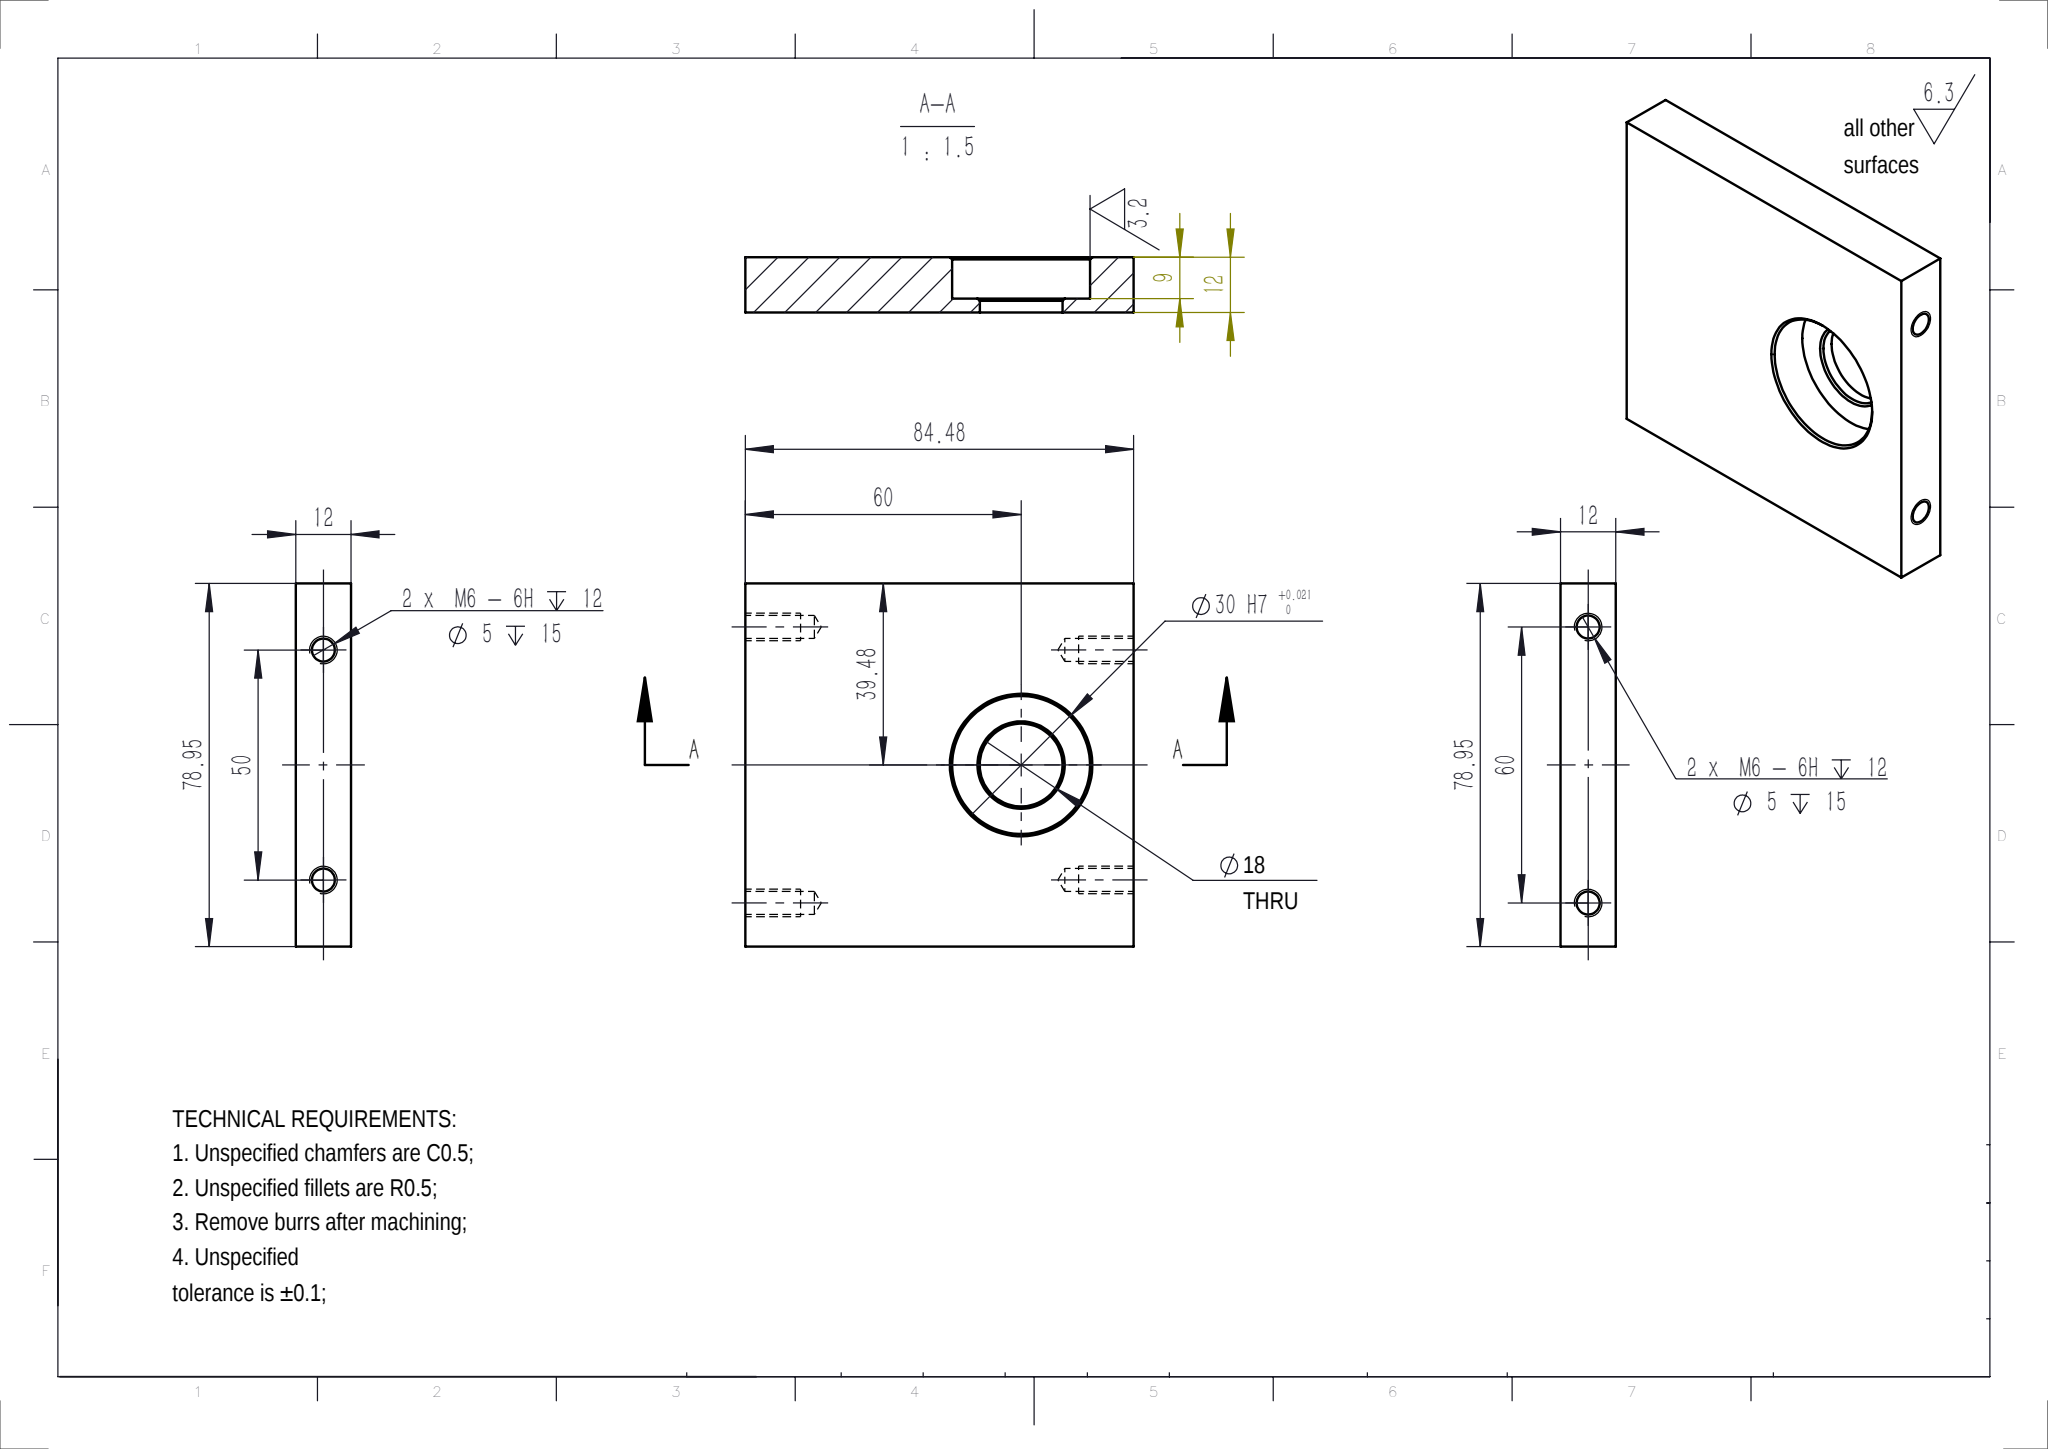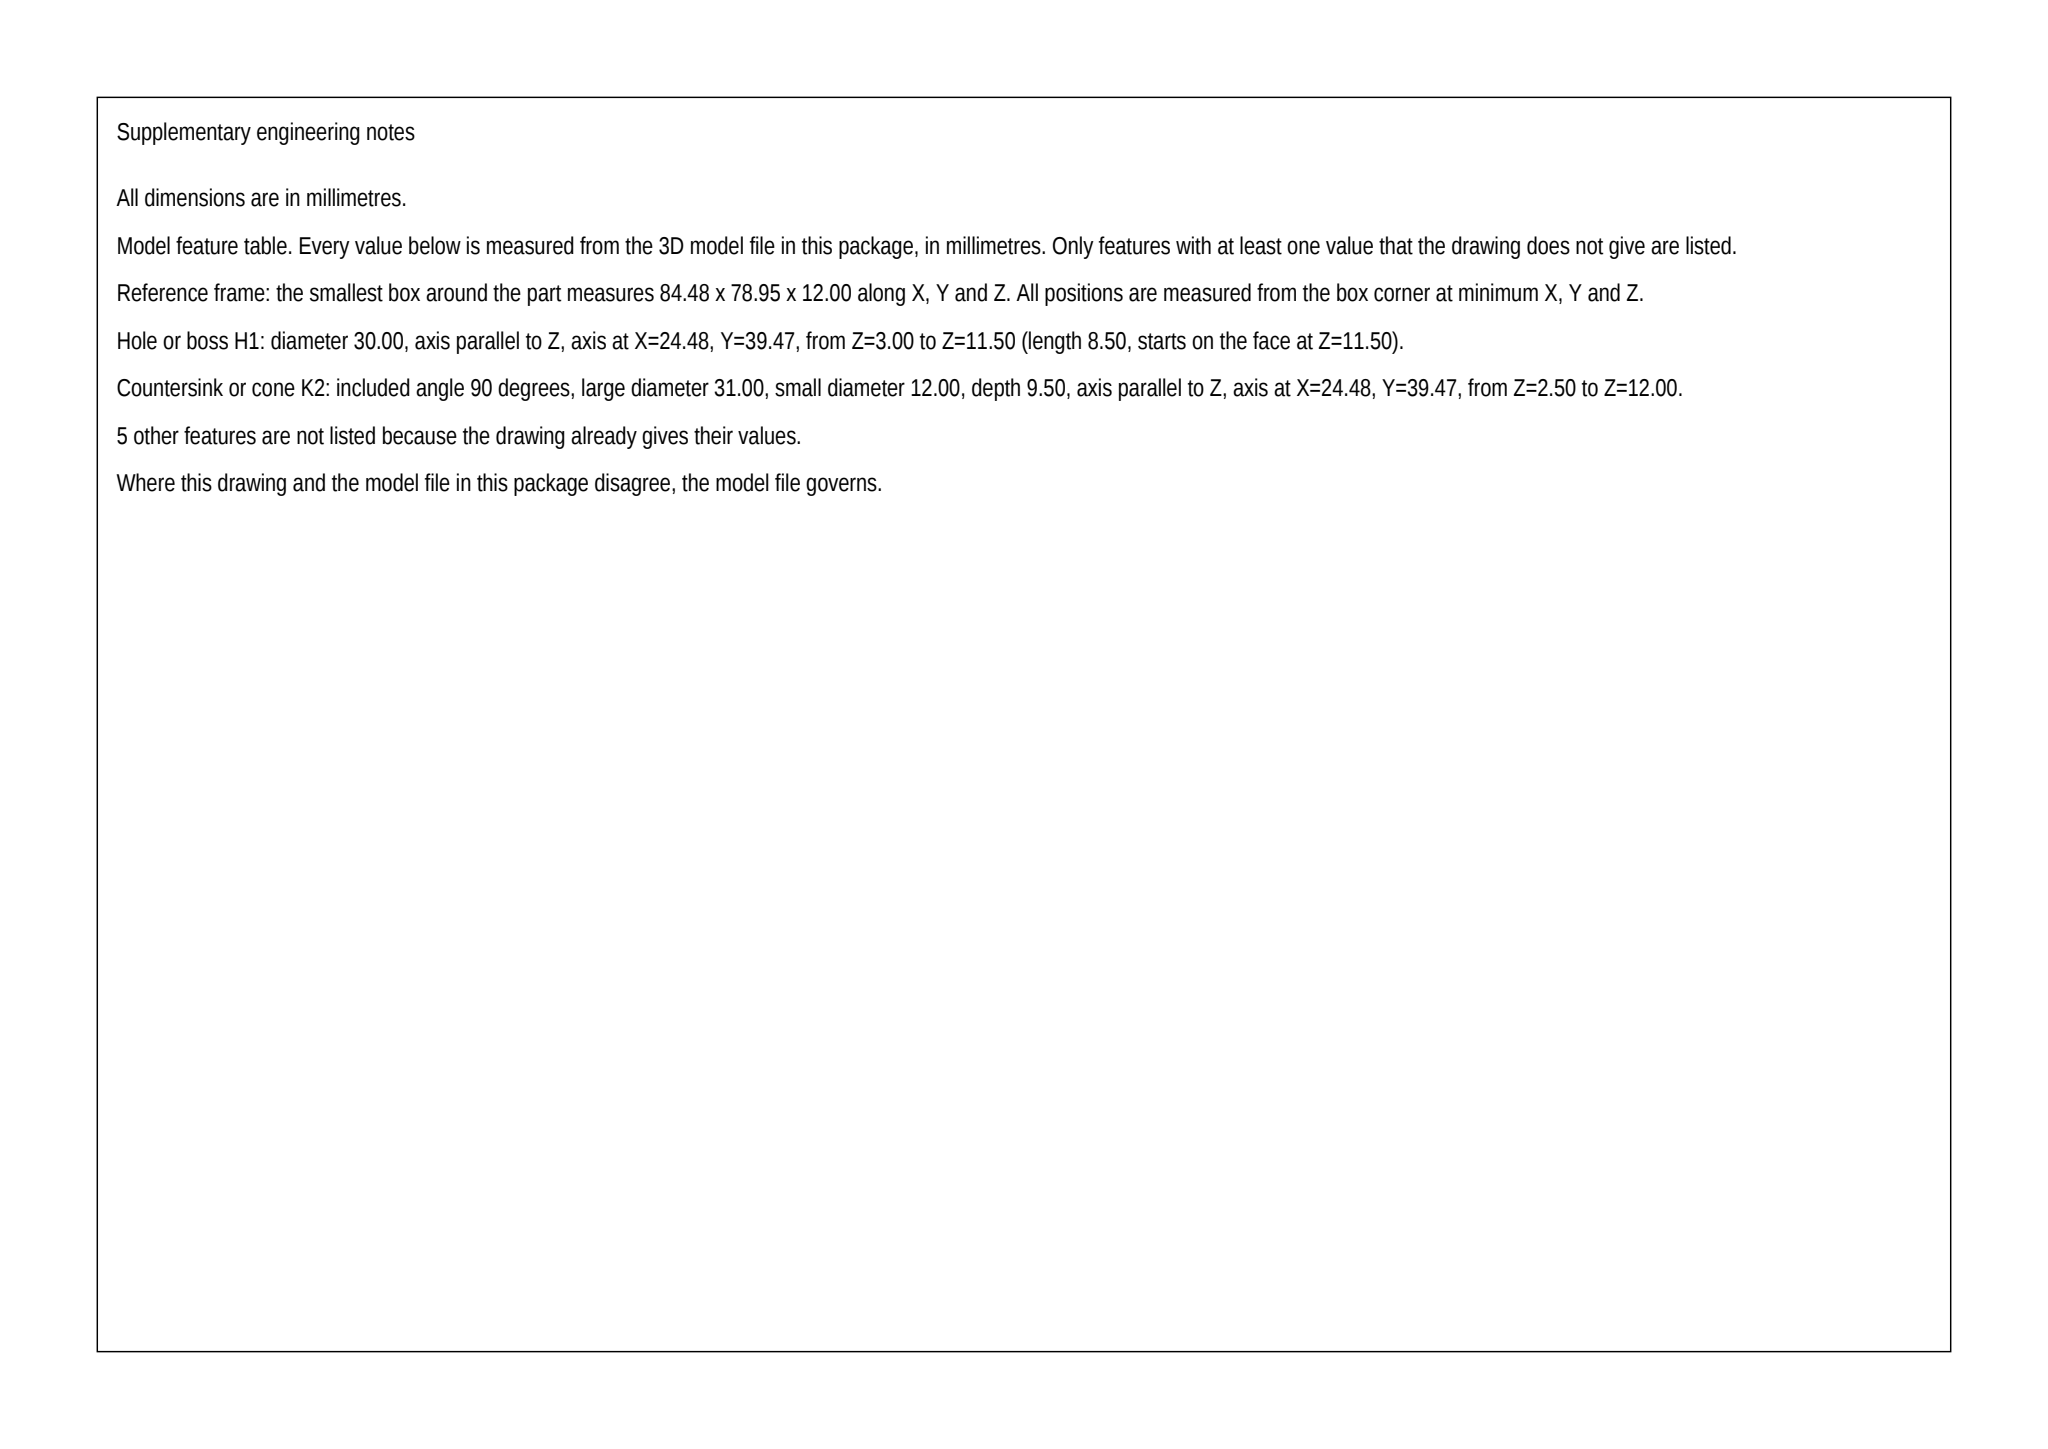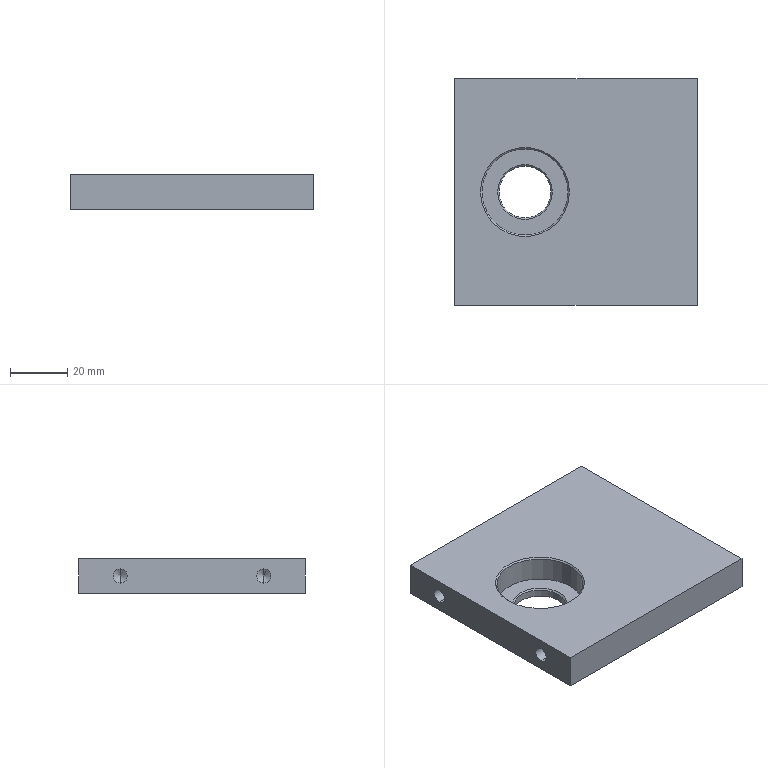Part | SolidWorks | mm | 1 solid | 31 faces | box 84.48 x 78.95 x 12 mm | volume 71675 mm3 | cone 12 | cylinder 12 | plane 7 | commonest cylinder face diameters 5 x8 18 x2 30 x2
build123d program:
from build123d import *

# Parameters (mm, degrees)
SKETCH1_W             = 84.48
SKETCH1_H             = 78.95
BOSS_EXTRUDE1_DEPTH   = 12
SKETCH2_R             = 15
CUT_EXTRUDE1_DEPTH    = 9
SKETCH3_R             = 9
CUT_EXTRUDE2_DEPTH    = 59.511
M6_TAPPED_HOLE1_D     = 5
M6_TAPPED_HOLE1_DEPTH = 15
M6_TAPPED_HOLE1_TIP   = 1.502
M6_TAPPED_HOLE2_D     = 5
M6_TAPPED_HOLE2_DEPTH = 15
M6_TAPPED_HOLE2_TIP   = 1.502
CHAMFER1_SIZE         = 0.5


with BuildPart() as part:
    # Sketch1 → Boss-Extrude1 (new body)
    with BuildSketch(Plane.XY):
        Rectangle(SKETCH1_W, SKETCH1_H)
    extrude(amount=BOSS_EXTRUDE1_DEPTH)

    # Sketch2 → Cut-Extrude1 (cut)
    with BuildSketch(Plane.XY.offset(12)):
        with Locations((-17.76, 0)):
            Circle(SKETCH2_R)
    extrude(amount=-CUT_EXTRUDE1_DEPTH, mode=Mode.SUBTRACT)

    # Sketch3 → Cut-Extrude2 (cut, through all)
    with BuildSketch(Plane.XY.offset(3)):
        with Locations((-17.76, 0)):
            Circle(SKETCH3_R)
    extrude(amount=-CUT_EXTRUDE2_DEPTH, mode=Mode.SUBTRACT)

    # M6 Tapped Hole1
    with Locations(Plane(origin=(42.24, 0, 0), x_dir=(0, 0, -1), z_dir=(1, 0, 0))):
        with Locations((-6, 30), (-6, -30)):
            Hole(M6_TAPPED_HOLE1_D / 2, depth=M6_TAPPED_HOLE1_DEPTH)
            with Locations((0, 0, -(M6_TAPPED_HOLE1_DEPTH + M6_TAPPED_HOLE1_TIP / 2))):  # 118° drill point
                Cone(0, M6_TAPPED_HOLE1_D / 2, M6_TAPPED_HOLE1_TIP, mode=Mode.SUBTRACT)

    # M6 Tapped Hole2
    with Locations(Plane.ZY.offset(42.24)):
        with Locations((6, 25), (6, -25)):
            Hole(M6_TAPPED_HOLE2_D / 2, depth=M6_TAPPED_HOLE2_DEPTH)
            with Locations((0, 0, -(M6_TAPPED_HOLE2_DEPTH + M6_TAPPED_HOLE2_TIP / 2))):  # 118° drill point
                Cone(0, M6_TAPPED_HOLE2_D / 2, M6_TAPPED_HOLE2_TIP, mode=Mode.SUBTRACT)

    # Chamfer1
    chamfer1_edges = [part.edges().sort_by_distance(p)[0] for p in [
        (-32.76, 0, 12),
        (-26.76, 0, 3),
    ]]
    chamfer(chamfer1_edges, length=CHAMFER1_SIZE)


solid = part.part
STEP:
#1=CARTESIAN_POINT('',(-26.76,0.,2.5));
#2=VERTEX_POINT('',#1);
#3=CARTESIAN_POINT('',(-8.76,0.,2.5));
#4=VERTEX_POINT('',#3);
#5=CARTESIAN_POINT('',(-17.76,0.,2.5));
#6=DIRECTION('',(0.,0.,1.));
#7=DIRECTION('',(1.,0.,0.));
#8=AXIS2_PLACEMENT_3D('',#5,#6,#7);
#9=CIRCLE('',#8,9.);
#10=EDGE_CURVE('',#2,#4,#9,.T.);
#11=ORIENTED_EDGE('',*,*,#10,.F.);
#12=CARTESIAN_POINT('',(-27.26,0.,3.));
#13=VERTEX_POINT('',#12);
#14=CARTESIAN_POINT('',(-26.76,0.,2.5));
#15=DIRECTION('',(-0.7071,0.,0.7071));
#16=VECTOR('',#15,1000.);
#17=LINE('',#14,#16);
#18=EDGE_CURVE('',#2,#13,#17,.T.);
#19=ORIENTED_EDGE('',*,*,#18,.T.);
#20=CARTESIAN_POINT('',(-8.26,0.,3.));
#21=VERTEX_POINT('',#20);
#22=CARTESIAN_POINT('',(-17.76,0.,3.));
#23=DIRECTION('',(0.,0.,-1.));
#24=DIRECTION('',(1.,0.,0.));
#25=AXIS2_PLACEMENT_3D('',#22,#23,#24);
#26=CIRCLE('',#25,9.5);
#27=EDGE_CURVE('',#21,#13,#26,.T.);
#28=ORIENTED_EDGE('',*,*,#27,.F.);
#29=CARTESIAN_POINT('',(-8.76,0.,2.5));
#30=DIRECTION('',(0.7071,0.,0.7071));
#31=VECTOR('',#30,1000.);
#32=LINE('',#29,#31);
#33=EDGE_CURVE('',#4,#21,#32,.T.);
#34=ORIENTED_EDGE('',*,*,#33,.F.);
#35=EDGE_LOOP('',(#11,#19,#28,#34));
#36=FACE_OUTER_BOUND('',#35,.T.);
#37=CARTESIAN_POINT('',(-17.76,0.,2.5));
#38=DIRECTION('',(0.,0.,1.));
#39=DIRECTION('',(1.,0.,0.));
#40=AXIS2_PLACEMENT_3D('',#37,#38,#39);
#41=CONICAL_SURFACE('',#40,9.,0.7854);
#42=ADVANCED_FACE('',(#36),#41,.F.);
#43=CARTESIAN_POINT('',(-32.76,0.,11.5));
#44=VERTEX_POINT('',#43);
#45=CARTESIAN_POINT('',(-2.76,0.,11.5));
#46=VERTEX_POINT('',#45);
#47=CARTESIAN_POINT('',(-17.76,0.,11.5));
#48=DIRECTION('',(0.,0.,1.));
#49=DIRECTION('',(1.,0.,0.));
#50=AXIS2_PLACEMENT_3D('',#47,#48,#49);
#51=CIRCLE('',#50,15.);
#52=EDGE_CURVE('',#44,#46,#51,.T.);
#53=ORIENTED_EDGE('',*,*,#52,.F.);
#54=CARTESIAN_POINT('',(-33.26,0.,12.));
#55=VERTEX_POINT('',#54);
#56=CARTESIAN_POINT('',(-32.76,0.,11.5));
#57=DIRECTION('',(-0.7071,0.,0.7071));
#58=VECTOR('',#57,1000.);
#59=LINE('',#56,#58);
#60=EDGE_CURVE('',#44,#55,#59,.T.);
#61=ORIENTED_EDGE('',*,*,#60,.T.);
#62=CARTESIAN_POINT('',(-2.26,0.,12.));
#63=VERTEX_POINT('',#62);
#64=CARTESIAN_POINT('',(-17.76,0.,12.));
#65=DIRECTION('',(0.,0.,-1.));
#66=DIRECTION('',(1.,0.,0.));
#67=AXIS2_PLACEMENT_3D('',#64,#65,#66);
#68=CIRCLE('',#67,15.5);
#69=EDGE_CURVE('',#63,#55,#68,.T.);
#70=ORIENTED_EDGE('',*,*,#69,.F.);
#71=CARTESIAN_POINT('',(-2.76,0.,11.5));
#72=DIRECTION('',(0.7071,0.,0.7071));
#73=VECTOR('',#72,1000.);
#74=LINE('',#71,#73);
#75=EDGE_CURVE('',#46,#63,#74,.T.);
#76=ORIENTED_EDGE('',*,*,#75,.F.);
#77=EDGE_LOOP('',(#53,#61,#70,#76));
#78=FACE_OUTER_BOUND('',#77,.T.);
#79=CARTESIAN_POINT('',(-17.76,0.,11.5));
#80=DIRECTION('',(0.,0.,1.));
#81=DIRECTION('',(1.,0.,0.));
#82=AXIS2_PLACEMENT_3D('',#79,#80,#81);
#83=CONICAL_SURFACE('',#82,15.,0.7854);
#84=ADVANCED_FACE('',(#78),#83,.F.);
#85=CARTESIAN_POINT('',(-27.24,25.,3.5));
#86=VERTEX_POINT('',#85);
#87=CARTESIAN_POINT('',(-27.24,25.,8.5));
#88=VERTEX_POINT('',#87);
#89=CARTESIAN_POINT('',(-27.24,25.,6.));
#90=DIRECTION('',(-1.,0.,0.));
#91=DIRECTION('',(0.,0.,1.));
#92=AXIS2_PLACEMENT_3D('',#89,#90,#91);
#93=CIRCLE('',#92,2.5);
#94=EDGE_CURVE('',#86,#88,#93,.T.);
#95=ORIENTED_EDGE('',*,*,#94,.F.);
#96=CARTESIAN_POINT('',(-42.24,25.,3.5));
#97=VERTEX_POINT('',#96);
#98=CARTESIAN_POINT('',(-42.24,25.,3.5));
#99=DIRECTION('',(-1.,0.,0.));
#100=VECTOR('',#99,1000.);
#101=LINE('',#98,#100);
#102=EDGE_CURVE('',#86,#97,#101,.T.);
#103=ORIENTED_EDGE('',*,*,#102,.T.);
#104=CARTESIAN_POINT('',(-42.24,25.,8.5));
#105=VERTEX_POINT('',#104);
#106=CARTESIAN_POINT('',(-42.24,25.,6.));
#107=DIRECTION('',(-1.,0.,0.));
#108=DIRECTION('',(0.,0.,1.));
#109=AXIS2_PLACEMENT_3D('',#106,#107,#108);
#110=CIRCLE('',#109,2.5);
#111=EDGE_CURVE('',#97,#105,#110,.T.);
#112=ORIENTED_EDGE('',*,*,#111,.T.);
#113=CARTESIAN_POINT('',(-42.24,25.,8.5));
#114=DIRECTION('',(-1.,0.,0.));
#115=VECTOR('',#114,1000.);
#116=LINE('',#113,#115);
#117=EDGE_CURVE('',#88,#105,#116,.T.);
#118=ORIENTED_EDGE('',*,*,#117,.F.);
#119=EDGE_LOOP('',(#95,#103,#112,#118));
#120=FACE_OUTER_BOUND('',#119,.T.);
#121=CARTESIAN_POINT('',(-42.24,25.,6.));
#122=DIRECTION('',(-1.,0.,0.));
#123=DIRECTION('',(0.,0.,1.));
#124=AXIS2_PLACEMENT_3D('',#121,#122,#123);
#125=CYLINDRICAL_SURFACE('',#124,2.5);
#126=ADVANCED_FACE('',(#120),#125,.F.);
#127=CARTESIAN_POINT('',(-25.738,25.,6.));
#128=VERTEX_POINT('',#127);
#129=CARTESIAN_POINT('',(-27.24,25.,8.5));
#130=DIRECTION('',(-0.515,0.,0.8572));
#131=VECTOR('',#130,1000.);
#132=LINE('',#129,#131);
#133=EDGE_CURVE('',#128,#88,#132,.T.);
#134=ORIENTED_EDGE('',*,*,#133,.F.);
#135=CARTESIAN_POINT('',(-27.24,25.,3.5));
#136=DIRECTION('',(-0.515,0.,-0.8572));
#137=VECTOR('',#136,1000.);
#138=LINE('',#135,#137);
#139=EDGE_CURVE('',#128,#86,#138,.T.);
#140=ORIENTED_EDGE('',*,*,#139,.T.);
#141=ORIENTED_EDGE('',*,*,#94,.T.);
#142=EDGE_LOOP('',(#134,#140,#141));
#143=FACE_OUTER_BOUND('',#142,.T.);
#144=CARTESIAN_POINT('',(-27.24,25.,6.));
#145=DIRECTION('',(-1.,0.,0.));
#146=DIRECTION('',(0.,0.,1.));
#147=AXIS2_PLACEMENT_3D('',#144,#145,#146);
#148=CONICAL_SURFACE('',#147,2.5,1.03);
#149=ADVANCED_FACE('',(#143),#148,.F.);
#150=CARTESIAN_POINT('',(-27.24,-25.,3.5));
#151=VERTEX_POINT('',#150);
#152=CARTESIAN_POINT('',(-27.24,-25.,8.5));
#153=VERTEX_POINT('',#152);
#154=CARTESIAN_POINT('',(-27.24,-25.,6.));
#155=DIRECTION('',(-1.,0.,0.));
#156=DIRECTION('',(0.,0.,1.));
#157=AXIS2_PLACEMENT_3D('',#154,#155,#156);
#158=CIRCLE('',#157,2.5);
#159=EDGE_CURVE('',#151,#153,#158,.T.);
#160=ORIENTED_EDGE('',*,*,#159,.F.);
#161=CARTESIAN_POINT('',(-42.24,-25.,3.5));
#162=VERTEX_POINT('',#161);
#163=CARTESIAN_POINT('',(-42.24,-25.,3.5));
#164=DIRECTION('',(-1.,0.,0.));
#165=VECTOR('',#164,1000.);
#166=LINE('',#163,#165);
#167=EDGE_CURVE('',#151,#162,#166,.T.);
#168=ORIENTED_EDGE('',*,*,#167,.T.);
#169=CARTESIAN_POINT('',(-42.24,-25.,8.5));
#170=VERTEX_POINT('',#169);
#171=CARTESIAN_POINT('',(-42.24,-25.,6.));
#172=DIRECTION('',(-1.,0.,0.));
#173=DIRECTION('',(0.,0.,1.));
#174=AXIS2_PLACEMENT_3D('',#171,#172,#173);
#175=CIRCLE('',#174,2.5);
#176=EDGE_CURVE('',#162,#170,#175,.T.);
#177=ORIENTED_EDGE('',*,*,#176,.T.);
#178=CARTESIAN_POINT('',(-42.24,-25.,8.5));
#179=DIRECTION('',(-1.,0.,0.));
#180=VECTOR('',#179,1000.);
#181=LINE('',#178,#180);
#182=EDGE_CURVE('',#153,#170,#181,.T.);
#183=ORIENTED_EDGE('',*,*,#182,.F.);
#184=EDGE_LOOP('',(#160,#168,#177,#183));
#185=FACE_OUTER_BOUND('',#184,.T.);
#186=CARTESIAN_POINT('',(-42.24,-25.,6.));
#187=DIRECTION('',(-1.,0.,0.));
#188=DIRECTION('',(0.,0.,1.));
#189=AXIS2_PLACEMENT_3D('',#186,#187,#188);
#190=CYLINDRICAL_SURFACE('',#189,2.5);
#191=ADVANCED_FACE('',(#185),#190,.F.);
#192=CARTESIAN_POINT('',(-25.738,-25.,6.));
#193=VERTEX_POINT('',#192);
#194=CARTESIAN_POINT('',(-27.24,-25.,8.5));
#195=DIRECTION('',(-0.515,0.,0.8572));
#196=VECTOR('',#195,1000.);
#197=LINE('',#194,#196);
#198=EDGE_CURVE('',#193,#153,#197,.T.);
#199=ORIENTED_EDGE('',*,*,#198,.F.);
#200=CARTESIAN_POINT('',(-27.24,-25.,3.5));
#201=DIRECTION('',(-0.515,0.,-0.8572));
#202=VECTOR('',#201,1000.);
#203=LINE('',#200,#202);
#204=EDGE_CURVE('',#193,#151,#203,.T.);
#205=ORIENTED_EDGE('',*,*,#204,.T.);
#206=ORIENTED_EDGE('',*,*,#159,.T.);
#207=EDGE_LOOP('',(#199,#205,#206));
#208=FACE_OUTER_BOUND('',#207,.T.);
#209=CARTESIAN_POINT('',(-27.24,-25.,6.));
#210=DIRECTION('',(-1.,0.,0.));
#211=DIRECTION('',(0.,0.,1.));
#212=AXIS2_PLACEMENT_3D('',#209,#210,#211);
#213=CONICAL_SURFACE('',#212,2.5,1.03);
#214=ADVANCED_FACE('',(#208),#213,.F.);
#215=CARTESIAN_POINT('',(27.24,30.,8.5));
#216=VERTEX_POINT('',#215);
#217=CARTESIAN_POINT('',(27.24,30.,3.5));
#218=VERTEX_POINT('',#217);
#219=CARTESIAN_POINT('',(27.24,30.,6.));
#220=DIRECTION('',(1.,0.,0.));
#221=DIRECTION('',(0.,0.,-1.));
#222=AXIS2_PLACEMENT_3D('',#219,#220,#221);
#223=CIRCLE('',#222,2.5);
#224=EDGE_CURVE('',#216,#218,#223,.T.);
#225=ORIENTED_EDGE('',*,*,#224,.F.);
#226=CARTESIAN_POINT('',(42.24,30.,8.5));
#227=VERTEX_POINT('',#226);
#228=CARTESIAN_POINT('',(42.24,30.,8.5));
#229=DIRECTION('',(1.,0.,0.));
#230=VECTOR('',#229,1000.);
#231=LINE('',#228,#230);
#232=EDGE_CURVE('',#216,#227,#231,.T.);
#233=ORIENTED_EDGE('',*,*,#232,.T.);
#234=CARTESIAN_POINT('',(42.24,30.,3.5));
#235=VERTEX_POINT('',#234);
#236=CARTESIAN_POINT('',(42.24,30.,6.));
#237=DIRECTION('',(1.,0.,0.));
#238=DIRECTION('',(0.,0.,-1.));
#239=AXIS2_PLACEMENT_3D('',#236,#237,#238);
#240=CIRCLE('',#239,2.5);
#241=EDGE_CURVE('',#227,#235,#240,.T.);
#242=ORIENTED_EDGE('',*,*,#241,.T.);
#243=CARTESIAN_POINT('',(42.24,30.,3.5));
#244=DIRECTION('',(1.,0.,0.));
#245=VECTOR('',#244,1000.);
#246=LINE('',#243,#245);
#247=EDGE_CURVE('',#218,#235,#246,.T.);
#248=ORIENTED_EDGE('',*,*,#247,.F.);
#249=EDGE_LOOP('',(#225,#233,#242,#248));
#250=FACE_OUTER_BOUND('',#249,.T.);
#251=CARTESIAN_POINT('',(42.24,30.,6.));
#252=DIRECTION('',(1.,0.,0.));
#253=DIRECTION('',(0.,0.,-1.));
#254=AXIS2_PLACEMENT_3D('',#251,#252,#253);
#255=CYLINDRICAL_SURFACE('',#254,2.5);
#256=ADVANCED_FACE('',(#250),#255,.F.);
#257=CARTESIAN_POINT('',(25.738,30.,6.));
#258=VERTEX_POINT('',#257);
#259=CARTESIAN_POINT('',(27.24,30.,3.5));
#260=DIRECTION('',(0.515,0.,-0.8572));
#261=VECTOR('',#260,1000.);
#262=LINE('',#259,#261);
#263=EDGE_CURVE('',#258,#218,#262,.T.);
#264=ORIENTED_EDGE('',*,*,#263,.F.);
#265=CARTESIAN_POINT('',(27.24,30.,8.5));
#266=DIRECTION('',(0.515,0.,0.8572));
#267=VECTOR('',#266,1000.);
#268=LINE('',#265,#267);
#269=EDGE_CURVE('',#258,#216,#268,.T.);
#270=ORIENTED_EDGE('',*,*,#269,.T.);
#271=ORIENTED_EDGE('',*,*,#224,.T.);
#272=EDGE_LOOP('',(#264,#270,#271));
#273=FACE_OUTER_BOUND('',#272,.T.);
#274=CARTESIAN_POINT('',(27.24,30.,6.));
#275=DIRECTION('',(1.,0.,0.));
#276=DIRECTION('',(0.,0.,-1.));
#277=AXIS2_PLACEMENT_3D('',#274,#275,#276);
#278=CONICAL_SURFACE('',#277,2.5,1.03);
#279=ADVANCED_FACE('',(#273),#278,.F.);
#280=CARTESIAN_POINT('',(27.24,-30.,8.5));
#281=VERTEX_POINT('',#280);
#282=CARTESIAN_POINT('',(27.24,-30.,3.5));
#283=VERTEX_POINT('',#282);
#284=CARTESIAN_POINT('',(27.24,-30.,6.));
#285=DIRECTION('',(1.,0.,0.));
#286=DIRECTION('',(0.,0.,-1.));
#287=AXIS2_PLACEMENT_3D('',#284,#285,#286);
#288=CIRCLE('',#287,2.5);
#289=EDGE_CURVE('',#281,#283,#288,.T.);
#290=ORIENTED_EDGE('',*,*,#289,.F.);
#291=CARTESIAN_POINT('',(42.24,-30.,8.5));
#292=VERTEX_POINT('',#291);
#293=CARTESIAN_POINT('',(42.24,-30.,8.5));
#294=DIRECTION('',(1.,0.,0.));
#295=VECTOR('',#294,1000.);
#296=LINE('',#293,#295);
#297=EDGE_CURVE('',#281,#292,#296,.T.);
#298=ORIENTED_EDGE('',*,*,#297,.T.);
#299=CARTESIAN_POINT('',(42.24,-30.,3.5));
#300=VERTEX_POINT('',#299);
#301=CARTESIAN_POINT('',(42.24,-30.,6.));
#302=DIRECTION('',(1.,0.,0.));
#303=DIRECTION('',(0.,0.,-1.));
#304=AXIS2_PLACEMENT_3D('',#301,#302,#303);
#305=CIRCLE('',#304,2.5);
#306=EDGE_CURVE('',#292,#300,#305,.T.);
#307=ORIENTED_EDGE('',*,*,#306,.T.);
#308=CARTESIAN_POINT('',(42.24,-30.,3.5));
#309=DIRECTION('',(1.,0.,0.));
#310=VECTOR('',#309,1000.);
#311=LINE('',#308,#310);
#312=EDGE_CURVE('',#283,#300,#311,.T.);
#313=ORIENTED_EDGE('',*,*,#312,.F.);
#314=EDGE_LOOP('',(#290,#298,#307,#313));
#315=FACE_OUTER_BOUND('',#314,.T.);
#316=CARTESIAN_POINT('',(42.24,-30.,6.));
#317=DIRECTION('',(1.,0.,0.));
#318=DIRECTION('',(0.,0.,-1.));
#319=AXIS2_PLACEMENT_3D('',#316,#317,#318);
#320=CYLINDRICAL_SURFACE('',#319,2.5);
#321=ADVANCED_FACE('',(#315),#320,.F.);
#322=CARTESIAN_POINT('',(25.738,-30.,6.));
#323=VERTEX_POINT('',#322);
#324=CARTESIAN_POINT('',(27.24,-30.,3.5));
#325=DIRECTION('',(0.515,0.,-0.8572));
#326=VECTOR('',#325,1000.);
#327=LINE('',#324,#326);
#328=EDGE_CURVE('',#323,#283,#327,.T.);
#329=ORIENTED_EDGE('',*,*,#328,.F.);
#330=CARTESIAN_POINT('',(27.24,-30.,8.5));
#331=DIRECTION('',(0.515,0.,0.8572));
#332=VECTOR('',#331,1000.);
#333=LINE('',#330,#332);
#334=EDGE_CURVE('',#323,#281,#333,.T.);
#335=ORIENTED_EDGE('',*,*,#334,.T.);
#336=ORIENTED_EDGE('',*,*,#289,.T.);
#337=EDGE_LOOP('',(#329,#335,#336));
#338=FACE_OUTER_BOUND('',#337,.T.);
#339=CARTESIAN_POINT('',(27.24,-30.,6.));
#340=DIRECTION('',(1.,0.,0.));
#341=DIRECTION('',(0.,0.,-1.));
#342=AXIS2_PLACEMENT_3D('',#339,#340,#341);
#343=CONICAL_SURFACE('',#342,2.5,1.03);
#344=ADVANCED_FACE('',(#338),#343,.F.);
#345=CARTESIAN_POINT('',(-26.76,0.,0.));
#346=VERTEX_POINT('',#345);
#347=CARTESIAN_POINT('',(-8.76,0.,0.));
#348=VERTEX_POINT('',#347);
#349=CARTESIAN_POINT('',(-17.76,0.,0.));
#350=DIRECTION('',(0.,0.,1.));
#351=DIRECTION('',(1.,0.,0.));
#352=AXIS2_PLACEMENT_3D('',#349,#350,#351);
#353=CIRCLE('',#352,9.);
#354=EDGE_CURVE('',#346,#348,#353,.T.);
#355=ORIENTED_EDGE('',*,*,#354,.F.);
#356=CARTESIAN_POINT('',(-26.76,0.,0.));
#357=DIRECTION('',(0.,0.,1.));
#358=VECTOR('',#357,1000.);
#359=LINE('',#356,#358);
#360=EDGE_CURVE('',#346,#2,#359,.T.);
#361=ORIENTED_EDGE('',*,*,#360,.T.);
#362=ORIENTED_EDGE('',*,*,#10,.T.);
#363=CARTESIAN_POINT('',(-8.76,0.,0.));
#364=DIRECTION('',(0.,0.,1.));
#365=VECTOR('',#364,1000.);
#366=LINE('',#363,#365);
#367=EDGE_CURVE('',#348,#4,#366,.T.);
#368=ORIENTED_EDGE('',*,*,#367,.F.);
#369=EDGE_LOOP('',(#355,#361,#362,#368));
#370=FACE_OUTER_BOUND('',#369,.T.);
#371=CARTESIAN_POINT('',(-17.76,0.,0.));
#372=DIRECTION('',(0.,0.,1.));
#373=DIRECTION('',(1.,0.,0.));
#374=AXIS2_PLACEMENT_3D('',#371,#372,#373);
#375=CYLINDRICAL_SURFACE('',#374,9.);
#376=ADVANCED_FACE('',(#370),#375,.F.);
#377=CARTESIAN_POINT('',(-32.76,0.,3.));
#378=VERTEX_POINT('',#377);
#379=CARTESIAN_POINT('',(-2.76,0.,3.));
#380=VERTEX_POINT('',#379);
#381=CARTESIAN_POINT('',(-17.76,0.,3.));
#382=DIRECTION('',(0.,0.,1.));
#383=DIRECTION('',(1.,0.,0.));
#384=AXIS2_PLACEMENT_3D('',#381,#382,#383);
#385=CIRCLE('',#384,15.);
#386=EDGE_CURVE('',#378,#380,#385,.T.);
#387=ORIENTED_EDGE('',*,*,#386,.F.);
#388=CARTESIAN_POINT('',(-32.76,0.,3.));
#389=DIRECTION('',(0.,0.,1.));
#390=VECTOR('',#389,1000.);
#391=LINE('',#388,#390);
#392=EDGE_CURVE('',#378,#44,#391,.T.);
#393=ORIENTED_EDGE('',*,*,#392,.T.);
#394=ORIENTED_EDGE('',*,*,#52,.T.);
#395=CARTESIAN_POINT('',(-2.76,0.,3.));
#396=DIRECTION('',(0.,0.,1.));
#397=VECTOR('',#396,1000.);
#398=LINE('',#395,#397);
#399=EDGE_CURVE('',#380,#46,#398,.T.);
#400=ORIENTED_EDGE('',*,*,#399,.F.);
#401=EDGE_LOOP('',(#387,#393,#394,#400));
#402=FACE_OUTER_BOUND('',#401,.T.);
#403=CARTESIAN_POINT('',(-17.76,0.,3.));
#404=DIRECTION('',(0.,0.,1.));
#405=DIRECTION('',(1.,0.,0.));
#406=AXIS2_PLACEMENT_3D('',#403,#404,#405);
#407=CYLINDRICAL_SURFACE('',#406,15.);
#408=ADVANCED_FACE('',(#402),#407,.F.);
#409=CARTESIAN_POINT('',(42.24,30.,6.));
#410=DIRECTION('',(1.,0.,0.));
#411=DIRECTION('',(0.,0.,-1.));
#412=AXIS2_PLACEMENT_3D('',#409,#410,#411);
#413=CIRCLE('',#412,2.5);
#414=EDGE_CURVE('',#235,#227,#413,.T.);
#415=ORIENTED_EDGE('',*,*,#414,.F.);
#416=ORIENTED_EDGE('',*,*,#241,.F.);
#417=EDGE_LOOP('',(#415,#416));
#418=FACE_BOUND('',#417,.T.);
#419=CARTESIAN_POINT('',(42.24,-30.,6.));
#420=DIRECTION('',(1.,0.,0.));
#421=DIRECTION('',(0.,0.,-1.));
#422=AXIS2_PLACEMENT_3D('',#419,#420,#421);
#423=CIRCLE('',#422,2.5);
#424=EDGE_CURVE('',#300,#292,#423,.T.);
#425=ORIENTED_EDGE('',*,*,#424,.F.);
#426=ORIENTED_EDGE('',*,*,#306,.F.);
#427=EDGE_LOOP('',(#425,#426));
#428=FACE_BOUND('',#427,.T.);
#429=CARTESIAN_POINT('',(42.24,-39.475,0.));
#430=VERTEX_POINT('',#429);
#431=CARTESIAN_POINT('',(42.24,39.475,0.));
#432=VERTEX_POINT('',#431);
#433=CARTESIAN_POINT('',(42.24,39.475,0.));
#434=DIRECTION('',(-0.,1.,0.));
#435=VECTOR('',#434,1000.);
#436=LINE('',#433,#435);
#437=EDGE_CURVE('',#430,#432,#436,.T.);
#438=ORIENTED_EDGE('',*,*,#437,.T.);
#439=CARTESIAN_POINT('',(42.24,39.475,12.));
#440=VERTEX_POINT('',#439);
#441=CARTESIAN_POINT('',(42.24,39.475,12.));
#442=DIRECTION('',(0.,0.,-1.));
#443=VECTOR('',#442,1000.);
#444=LINE('',#441,#443);
#445=EDGE_CURVE('',#440,#432,#444,.T.);
#446=ORIENTED_EDGE('',*,*,#445,.F.);
#447=CARTESIAN_POINT('',(42.24,-39.475,12.));
#448=VERTEX_POINT('',#447);
#449=CARTESIAN_POINT('',(42.24,39.475,12.));
#450=DIRECTION('',(-0.,1.,0.));
#451=VECTOR('',#450,1000.);
#452=LINE('',#449,#451);
#453=EDGE_CURVE('',#448,#440,#452,.T.);
#454=ORIENTED_EDGE('',*,*,#453,.F.);
#455=CARTESIAN_POINT('',(42.24,-39.475,12.));
#456=DIRECTION('',(0.,0.,-1.));
#457=VECTOR('',#456,1000.);
#458=LINE('',#455,#457);
#459=EDGE_CURVE('',#448,#430,#458,.T.);
#460=ORIENTED_EDGE('',*,*,#459,.T.);
#461=EDGE_LOOP('',(#438,#446,#454,#460));
#462=FACE_OUTER_BOUND('',#461,.T.);
#463=CARTESIAN_POINT('',(42.24,39.475,12.));
#464=DIRECTION('',(-1.,-0.,0.));
#465=DIRECTION('',(0.,-1.,0.));
#466=AXIS2_PLACEMENT_3D('',#463,#464,#465);
#467=PLANE('',#466);
#468=ADVANCED_FACE('',(#418,#428,#462),#467,.F.);
#469=CARTESIAN_POINT('',(-42.24,39.475,0.));
#470=VERTEX_POINT('',#469);
#471=CARTESIAN_POINT('',(-42.24,39.475,0.));
#472=DIRECTION('',(-1.,0.,0.));
#473=VECTOR('',#472,1000.);
#474=LINE('',#471,#473);
#475=EDGE_CURVE('',#432,#470,#474,.T.);
#476=ORIENTED_EDGE('',*,*,#475,.T.);
#477=CARTESIAN_POINT('',(-42.24,39.475,12.));
#478=VERTEX_POINT('',#477);
#479=CARTESIAN_POINT('',(-42.24,39.475,12.));
#480=DIRECTION('',(0.,0.,-1.));
#481=VECTOR('',#480,1000.);
#482=LINE('',#479,#481);
#483=EDGE_CURVE('',#478,#470,#482,.T.);
#484=ORIENTED_EDGE('',*,*,#483,.F.);
#485=CARTESIAN_POINT('',(-42.24,39.475,12.));
#486=DIRECTION('',(-1.,0.,0.));
#487=VECTOR('',#486,1000.);
#488=LINE('',#485,#487);
#489=EDGE_CURVE('',#440,#478,#488,.T.);
#490=ORIENTED_EDGE('',*,*,#489,.F.);
#491=ORIENTED_EDGE('',*,*,#445,.T.);
#492=EDGE_LOOP('',(#476,#484,#490,#491));
#493=FACE_OUTER_BOUND('',#492,.T.);
#494=CARTESIAN_POINT('',(-42.24,39.475,12.));
#495=DIRECTION('',(0.,-1.,0.));
#496=DIRECTION('',(0.,0.,-1.));
#497=AXIS2_PLACEMENT_3D('',#494,#495,#496);
#498=PLANE('',#497);
#499=ADVANCED_FACE('',(#493),#498,.F.);
#500=CARTESIAN_POINT('',(-42.24,25.,6.));
#501=DIRECTION('',(-1.,0.,0.));
#502=DIRECTION('',(0.,0.,1.));
#503=AXIS2_PLACEMENT_3D('',#500,#501,#502);
#504=CIRCLE('',#503,2.5);
#505=EDGE_CURVE('',#105,#97,#504,.T.);
#506=ORIENTED_EDGE('',*,*,#505,.F.);
#507=ORIENTED_EDGE('',*,*,#111,.F.);
#508=EDGE_LOOP('',(#506,#507));
#509=FACE_BOUND('',#508,.T.);
#510=CARTESIAN_POINT('',(-42.24,-25.,6.));
#511=DIRECTION('',(-1.,0.,0.));
#512=DIRECTION('',(0.,0.,1.));
#513=AXIS2_PLACEMENT_3D('',#510,#511,#512);
#514=CIRCLE('',#513,2.5);
#515=EDGE_CURVE('',#170,#162,#514,.T.);
#516=ORIENTED_EDGE('',*,*,#515,.F.);
#517=ORIENTED_EDGE('',*,*,#176,.F.);
#518=EDGE_LOOP('',(#516,#517));
#519=FACE_BOUND('',#518,.T.);
#520=CARTESIAN_POINT('',(-42.24,-39.475,0.));
#521=VERTEX_POINT('',#520);
#522=CARTESIAN_POINT('',(-42.24,39.475,0.));
#523=DIRECTION('',(0.,-1.,0.));
#524=VECTOR('',#523,1000.);
#525=LINE('',#522,#524);
#526=EDGE_CURVE('',#470,#521,#525,.T.);
#527=ORIENTED_EDGE('',*,*,#526,.T.);
#528=CARTESIAN_POINT('',(-42.24,-39.475,12.));
#529=VERTEX_POINT('',#528);
#530=CARTESIAN_POINT('',(-42.24,-39.475,12.));
#531=DIRECTION('',(0.,0.,-1.));
#532=VECTOR('',#531,1000.);
#533=LINE('',#530,#532);
#534=EDGE_CURVE('',#529,#521,#533,.T.);
#535=ORIENTED_EDGE('',*,*,#534,.F.);
#536=CARTESIAN_POINT('',(-42.24,39.475,12.));
#537=DIRECTION('',(0.,-1.,0.));
#538=VECTOR('',#537,1000.);
#539=LINE('',#536,#538);
#540=EDGE_CURVE('',#478,#529,#539,.T.);
#541=ORIENTED_EDGE('',*,*,#540,.F.);
#542=ORIENTED_EDGE('',*,*,#483,.T.);
#543=EDGE_LOOP('',(#527,#535,#541,#542));
#544=FACE_OUTER_BOUND('',#543,.T.);
#545=CARTESIAN_POINT('',(-42.24,39.475,12.));
#546=DIRECTION('',(1.,0.,0.));
#547=DIRECTION('',(-0.,1.,0.));
#548=AXIS2_PLACEMENT_3D('',#545,#546,#547);
#549=PLANE('',#548);
#550=ADVANCED_FACE('',(#509,#519,#544),#549,.F.);
#551=CARTESIAN_POINT('',(-42.24,-39.475,0.));
#552=DIRECTION('',(1.,0.,0.));
#553=VECTOR('',#552,1000.);
#554=LINE('',#551,#553);
#555=EDGE_CURVE('',#521,#430,#554,.T.);
#556=ORIENTED_EDGE('',*,*,#555,.T.);
#557=ORIENTED_EDGE('',*,*,#459,.F.);
#558=CARTESIAN_POINT('',(-42.24,-39.475,12.));
#559=DIRECTION('',(1.,0.,0.));
#560=VECTOR('',#559,1000.);
#561=LINE('',#558,#560);
#562=EDGE_CURVE('',#529,#448,#561,.T.);
#563=ORIENTED_EDGE('',*,*,#562,.F.);
#564=ORIENTED_EDGE('',*,*,#534,.T.);
#565=EDGE_LOOP('',(#556,#557,#563,#564));
#566=FACE_OUTER_BOUND('',#565,.T.);
#567=CARTESIAN_POINT('',(-42.24,-39.475,12.));
#568=DIRECTION('',(0.,1.,0.));
#569=DIRECTION('',(0.,0.,1.));
#570=AXIS2_PLACEMENT_3D('',#567,#568,#569);
#571=PLANE('',#570);
#572=ADVANCED_FACE('',(#566),#571,.F.);
#573=ORIENTED_EDGE('',*,*,#69,.T.);
#574=CARTESIAN_POINT('',(-17.76,0.,12.));
#575=DIRECTION('',(0.,0.,-1.));
#576=DIRECTION('',(1.,0.,0.));
#577=AXIS2_PLACEMENT_3D('',#574,#575,#576);
#578=CIRCLE('',#577,15.5);
#579=EDGE_CURVE('',#55,#63,#578,.T.);
#580=ORIENTED_EDGE('',*,*,#579,.T.);
#581=EDGE_LOOP('',(#573,#580));
#582=FACE_BOUND('',#581,.T.);
#583=ORIENTED_EDGE('',*,*,#453,.T.);
#584=ORIENTED_EDGE('',*,*,#489,.T.);
#585=ORIENTED_EDGE('',*,*,#540,.T.);
#586=ORIENTED_EDGE('',*,*,#562,.T.);
#587=EDGE_LOOP('',(#583,#584,#585,#586));
#588=FACE_OUTER_BOUND('',#587,.T.);
#589=CARTESIAN_POINT('',(0.,0.,12.));
#590=DIRECTION('',(0.,0.,1.));
#591=DIRECTION('',(1.,0.,0.));
#592=AXIS2_PLACEMENT_3D('',#589,#590,#591);
#593=PLANE('',#592);
#594=ADVANCED_FACE('',(#582,#588),#593,.T.);
#595=CARTESIAN_POINT('',(-17.76,0.,0.));
#596=DIRECTION('',(0.,0.,1.));
#597=DIRECTION('',(1.,0.,0.));
#598=AXIS2_PLACEMENT_3D('',#595,#596,#597);
#599=CIRCLE('',#598,9.);
#600=EDGE_CURVE('',#348,#346,#599,.T.);
#601=ORIENTED_EDGE('',*,*,#600,.T.);
#602=ORIENTED_EDGE('',*,*,#354,.T.);
#603=EDGE_LOOP('',(#601,#602));
#604=FACE_BOUND('',#603,.T.);
#605=ORIENTED_EDGE('',*,*,#437,.F.);
#606=ORIENTED_EDGE('',*,*,#555,.F.);
#607=ORIENTED_EDGE('',*,*,#526,.F.);
#608=ORIENTED_EDGE('',*,*,#475,.F.);
#609=EDGE_LOOP('',(#605,#606,#607,#608));
#610=FACE_OUTER_BOUND('',#609,.T.);
#611=CARTESIAN_POINT('',(0.,0.,0.));
#612=DIRECTION('',(0.,0.,1.));
#613=DIRECTION('',(1.,0.,0.));
#614=AXIS2_PLACEMENT_3D('',#611,#612,#613);
#615=PLANE('',#614);
#616=ADVANCED_FACE('',(#604,#610),#615,.F.);
#617=ORIENTED_EDGE('',*,*,#392,.F.);
#618=CARTESIAN_POINT('',(-17.76,0.,3.));
#619=DIRECTION('',(0.,0.,1.));
#620=DIRECTION('',(1.,0.,0.));
#621=AXIS2_PLACEMENT_3D('',#618,#619,#620);
#622=CIRCLE('',#621,15.);
#623=EDGE_CURVE('',#380,#378,#622,.T.);
#624=ORIENTED_EDGE('',*,*,#623,.F.);
#625=ORIENTED_EDGE('',*,*,#399,.T.);
#626=CARTESIAN_POINT('',(-17.76,0.,11.5));
#627=DIRECTION('',(0.,0.,1.));
#628=DIRECTION('',(1.,0.,0.));
#629=AXIS2_PLACEMENT_3D('',#626,#627,#628);
#630=CIRCLE('',#629,15.);
#631=EDGE_CURVE('',#46,#44,#630,.T.);
#632=ORIENTED_EDGE('',*,*,#631,.T.);
#633=EDGE_LOOP('',(#617,#624,#625,#632));
#634=FACE_OUTER_BOUND('',#633,.T.);
#635=CARTESIAN_POINT('',(-17.76,0.,3.));
#636=DIRECTION('',(0.,0.,1.));
#637=DIRECTION('',(1.,0.,0.));
#638=AXIS2_PLACEMENT_3D('',#635,#636,#637);
#639=CYLINDRICAL_SURFACE('',#638,15.);
#640=ADVANCED_FACE('',(#634),#639,.F.);
#641=ORIENTED_EDGE('',*,*,#27,.T.);
#642=CARTESIAN_POINT('',(-17.76,0.,3.));
#643=DIRECTION('',(0.,0.,-1.));
#644=DIRECTION('',(1.,0.,0.));
#645=AXIS2_PLACEMENT_3D('',#642,#643,#644);
#646=CIRCLE('',#645,9.5);
#647=EDGE_CURVE('',#13,#21,#646,.T.);
#648=ORIENTED_EDGE('',*,*,#647,.T.);
#649=EDGE_LOOP('',(#641,#648));
#650=FACE_BOUND('',#649,.T.);
#651=ORIENTED_EDGE('',*,*,#623,.T.);
#652=ORIENTED_EDGE('',*,*,#386,.T.);
#653=EDGE_LOOP('',(#651,#652));
#654=FACE_OUTER_BOUND('',#653,.T.);
#655=CARTESIAN_POINT('',(-17.76,0.,3.));
#656=DIRECTION('',(0.,0.,1.));
#657=DIRECTION('',(1.,0.,0.));
#658=AXIS2_PLACEMENT_3D('',#655,#656,#657);
#659=PLANE('',#658);
#660=ADVANCED_FACE('',(#650,#654),#659,.T.);
#661=ORIENTED_EDGE('',*,*,#360,.F.);
#662=ORIENTED_EDGE('',*,*,#600,.F.);
#663=ORIENTED_EDGE('',*,*,#367,.T.);
#664=CARTESIAN_POINT('',(-17.76,0.,2.5));
#665=DIRECTION('',(0.,0.,1.));
#666=DIRECTION('',(1.,0.,0.));
#667=AXIS2_PLACEMENT_3D('',#664,#665,#666);
#668=CIRCLE('',#667,9.);
#669=EDGE_CURVE('',#4,#2,#668,.T.);
#670=ORIENTED_EDGE('',*,*,#669,.T.);
#671=EDGE_LOOP('',(#661,#662,#663,#670));
#672=FACE_OUTER_BOUND('',#671,.T.);
#673=CARTESIAN_POINT('',(-17.76,0.,0.));
#674=DIRECTION('',(0.,0.,1.));
#675=DIRECTION('',(1.,0.,0.));
#676=AXIS2_PLACEMENT_3D('',#673,#674,#675);
#677=CYLINDRICAL_SURFACE('',#676,9.);
#678=ADVANCED_FACE('',(#672),#677,.F.);
#679=ORIENTED_EDGE('',*,*,#334,.F.);
#680=ORIENTED_EDGE('',*,*,#328,.T.);
#681=CARTESIAN_POINT('',(27.24,-30.,6.));
#682=DIRECTION('',(1.,0.,0.));
#683=DIRECTION('',(0.,0.,-1.));
#684=AXIS2_PLACEMENT_3D('',#681,#682,#683);
#685=CIRCLE('',#684,2.5);
#686=EDGE_CURVE('',#283,#281,#685,.T.);
#687=ORIENTED_EDGE('',*,*,#686,.T.);
#688=EDGE_LOOP('',(#679,#680,#687));
#689=FACE_OUTER_BOUND('',#688,.T.);
#690=CARTESIAN_POINT('',(27.24,-30.,6.));
#691=DIRECTION('',(1.,0.,0.));
#692=DIRECTION('',(0.,0.,-1.));
#693=AXIS2_PLACEMENT_3D('',#690,#691,#692);
#694=CONICAL_SURFACE('',#693,2.5,1.03);
#695=ADVANCED_FACE('',(#689),#694,.F.);
#696=ORIENTED_EDGE('',*,*,#297,.F.);
#697=ORIENTED_EDGE('',*,*,#686,.F.);
#698=ORIENTED_EDGE('',*,*,#312,.T.);
#699=ORIENTED_EDGE('',*,*,#424,.T.);
#700=EDGE_LOOP('',(#696,#697,#698,#699));
#701=FACE_OUTER_BOUND('',#700,.T.);
#702=CARTESIAN_POINT('',(42.24,-30.,6.));
#703=DIRECTION('',(1.,0.,0.));
#704=DIRECTION('',(0.,0.,-1.));
#705=AXIS2_PLACEMENT_3D('',#702,#703,#704);
#706=CYLINDRICAL_SURFACE('',#705,2.5);
#707=ADVANCED_FACE('',(#701),#706,.F.);
#708=ORIENTED_EDGE('',*,*,#269,.F.);
#709=ORIENTED_EDGE('',*,*,#263,.T.);
#710=CARTESIAN_POINT('',(27.24,30.,6.));
#711=DIRECTION('',(1.,0.,0.));
#712=DIRECTION('',(0.,0.,-1.));
#713=AXIS2_PLACEMENT_3D('',#710,#711,#712);
#714=CIRCLE('',#713,2.5);
#715=EDGE_CURVE('',#218,#216,#714,.T.);
#716=ORIENTED_EDGE('',*,*,#715,.T.);
#717=EDGE_LOOP('',(#708,#709,#716));
#718=FACE_OUTER_BOUND('',#717,.T.);
#719=CARTESIAN_POINT('',(27.24,30.,6.));
#720=DIRECTION('',(1.,0.,0.));
#721=DIRECTION('',(0.,0.,-1.));
#722=AXIS2_PLACEMENT_3D('',#719,#720,#721);
#723=CONICAL_SURFACE('',#722,2.5,1.03);
#724=ADVANCED_FACE('',(#718),#723,.F.);
#725=ORIENTED_EDGE('',*,*,#232,.F.);
#726=ORIENTED_EDGE('',*,*,#715,.F.);
#727=ORIENTED_EDGE('',*,*,#247,.T.);
#728=ORIENTED_EDGE('',*,*,#414,.T.);
#729=EDGE_LOOP('',(#725,#726,#727,#728));
#730=FACE_OUTER_BOUND('',#729,.T.);
#731=CARTESIAN_POINT('',(42.24,30.,6.));
#732=DIRECTION('',(1.,0.,0.));
#733=DIRECTION('',(0.,0.,-1.));
#734=AXIS2_PLACEMENT_3D('',#731,#732,#733);
#735=CYLINDRICAL_SURFACE('',#734,2.5);
#736=ADVANCED_FACE('',(#730),#735,.F.);
#737=ORIENTED_EDGE('',*,*,#204,.F.);
#738=ORIENTED_EDGE('',*,*,#198,.T.);
#739=CARTESIAN_POINT('',(-27.24,-25.,6.));
#740=DIRECTION('',(-1.,0.,0.));
#741=DIRECTION('',(0.,0.,1.));
#742=AXIS2_PLACEMENT_3D('',#739,#740,#741);
#743=CIRCLE('',#742,2.5);
#744=EDGE_CURVE('',#153,#151,#743,.T.);
#745=ORIENTED_EDGE('',*,*,#744,.T.);
#746=EDGE_LOOP('',(#737,#738,#745));
#747=FACE_OUTER_BOUND('',#746,.T.);
#748=CARTESIAN_POINT('',(-27.24,-25.,6.));
#749=DIRECTION('',(-1.,0.,0.));
#750=DIRECTION('',(0.,0.,1.));
#751=AXIS2_PLACEMENT_3D('',#748,#749,#750);
#752=CONICAL_SURFACE('',#751,2.5,1.03);
#753=ADVANCED_FACE('',(#747),#752,.F.);
#754=ORIENTED_EDGE('',*,*,#167,.F.);
#755=ORIENTED_EDGE('',*,*,#744,.F.);
#756=ORIENTED_EDGE('',*,*,#182,.T.);
#757=ORIENTED_EDGE('',*,*,#515,.T.);
#758=EDGE_LOOP('',(#754,#755,#756,#757));
#759=FACE_OUTER_BOUND('',#758,.T.);
#760=CARTESIAN_POINT('',(-42.24,-25.,6.));
#761=DIRECTION('',(-1.,0.,0.));
#762=DIRECTION('',(0.,0.,1.));
#763=AXIS2_PLACEMENT_3D('',#760,#761,#762);
#764=CYLINDRICAL_SURFACE('',#763,2.5);
#765=ADVANCED_FACE('',(#759),#764,.F.);
#766=ORIENTED_EDGE('',*,*,#139,.F.);
#767=ORIENTED_EDGE('',*,*,#133,.T.);
#768=CARTESIAN_POINT('',(-27.24,25.,6.));
#769=DIRECTION('',(-1.,0.,0.));
#770=DIRECTION('',(0.,0.,1.));
#771=AXIS2_PLACEMENT_3D('',#768,#769,#770);
#772=CIRCLE('',#771,2.5);
#773=EDGE_CURVE('',#88,#86,#772,.T.);
#774=ORIENTED_EDGE('',*,*,#773,.T.);
#775=EDGE_LOOP('',(#766,#767,#774));
#776=FACE_OUTER_BOUND('',#775,.T.);
#777=CARTESIAN_POINT('',(-27.24,25.,6.));
#778=DIRECTION('',(-1.,0.,0.));
#779=DIRECTION('',(0.,0.,1.));
#780=AXIS2_PLACEMENT_3D('',#777,#778,#779);
#781=CONICAL_SURFACE('',#780,2.5,1.03);
#782=ADVANCED_FACE('',(#776),#781,.F.);
#783=ORIENTED_EDGE('',*,*,#102,.F.);
#784=ORIENTED_EDGE('',*,*,#773,.F.);
#785=ORIENTED_EDGE('',*,*,#117,.T.);
#786=ORIENTED_EDGE('',*,*,#505,.T.);
#787=EDGE_LOOP('',(#783,#784,#785,#786));
#788=FACE_OUTER_BOUND('',#787,.T.);
#789=CARTESIAN_POINT('',(-42.24,25.,6.));
#790=DIRECTION('',(-1.,0.,0.));
#791=DIRECTION('',(0.,0.,1.));
#792=AXIS2_PLACEMENT_3D('',#789,#790,#791);
#793=CYLINDRICAL_SURFACE('',#792,2.5);
#794=ADVANCED_FACE('',(#788),#793,.F.);
#795=ORIENTED_EDGE('',*,*,#60,.F.);
#796=ORIENTED_EDGE('',*,*,#631,.F.);
#797=ORIENTED_EDGE('',*,*,#75,.T.);
#798=ORIENTED_EDGE('',*,*,#579,.F.);
#799=EDGE_LOOP('',(#795,#796,#797,#798));
#800=FACE_OUTER_BOUND('',#799,.T.);
#801=CARTESIAN_POINT('',(-17.76,0.,11.5));
#802=DIRECTION('',(0.,0.,1.));
#803=DIRECTION('',(1.,0.,0.));
#804=AXIS2_PLACEMENT_3D('',#801,#802,#803);
#805=CONICAL_SURFACE('',#804,15.,0.7854);
#806=ADVANCED_FACE('',(#800),#805,.F.);
#807=ORIENTED_EDGE('',*,*,#18,.F.);
#808=ORIENTED_EDGE('',*,*,#669,.F.);
#809=ORIENTED_EDGE('',*,*,#33,.T.);
#810=ORIENTED_EDGE('',*,*,#647,.F.);
#811=EDGE_LOOP('',(#807,#808,#809,#810));
#812=FACE_OUTER_BOUND('',#811,.T.);
#813=CARTESIAN_POINT('',(-17.76,0.,2.5));
#814=DIRECTION('',(0.,0.,1.));
#815=DIRECTION('',(1.,0.,0.));
#816=AXIS2_PLACEMENT_3D('',#813,#814,#815);
#817=CONICAL_SURFACE('',#816,9.,0.7854);
#818=ADVANCED_FACE('',(#812),#817,.F.);
#819=CLOSED_SHELL('',(#42,#84,#126,#149,#191,#214,#256,#279,#321,#344,#376,#408,#468,#499,#550,#572,#594,#616,#640,#660,#678,#695,#707,#724,#736,#753,#765,#782,#794,#806,#818));
#820=MANIFOLD_SOLID_BREP('',#819);
#821=CARTESIAN_POINT('',(0.,0.,0.));
#822=DIRECTION('',(0.,0.,1.));
#823=DIRECTION('',(1.,0.,0.));
#824=AXIS2_PLACEMENT_3D('',#821,#822,#823);
#825=(LENGTH_UNIT()NAMED_UNIT(*)SI_UNIT(.MILLI.,.METRE.));
#826=UNCERTAINTY_MEASURE_WITH_UNIT(LENGTH_MEASURE(0.00001),#825,'','');
#827=(NAMED_UNIT(*)PLANE_ANGLE_UNIT()SI_UNIT($,.RADIAN.));
#828=(NAMED_UNIT(*)SI_UNIT($,.STERADIAN.)SOLID_ANGLE_UNIT());
#829=(GEOMETRIC_REPRESENTATION_CONTEXT(3)GLOBAL_UNCERTAINTY_ASSIGNED_CONTEXT((#826))GLOBAL_UNIT_ASSIGNED_CONTEXT((#825,#827,#828))REPRESENTATION_CONTEXT('',''));
#830=ADVANCED_BREP_SHAPE_REPRESENTATION('',(#820,#824),#829);